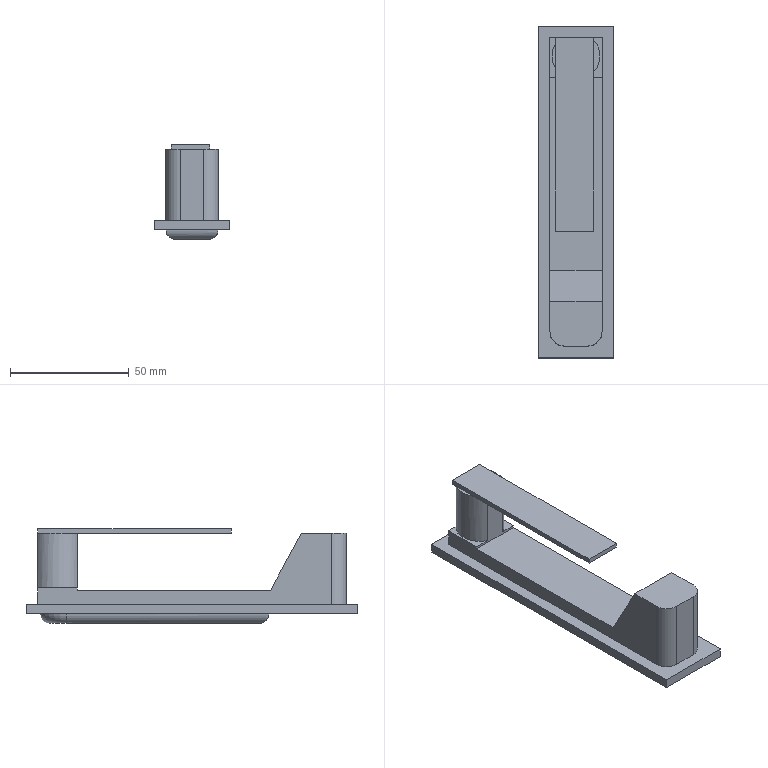Component | SolidWorks | RightRearDoor-1_Lock818-1 | 1 solid | 45 faces | volume 64552 mm3 | plane 35 | cylinder 9 | torus 1 | commonest cylinder face diameters 8 x3 22 x2 20.166 x2 12 x2